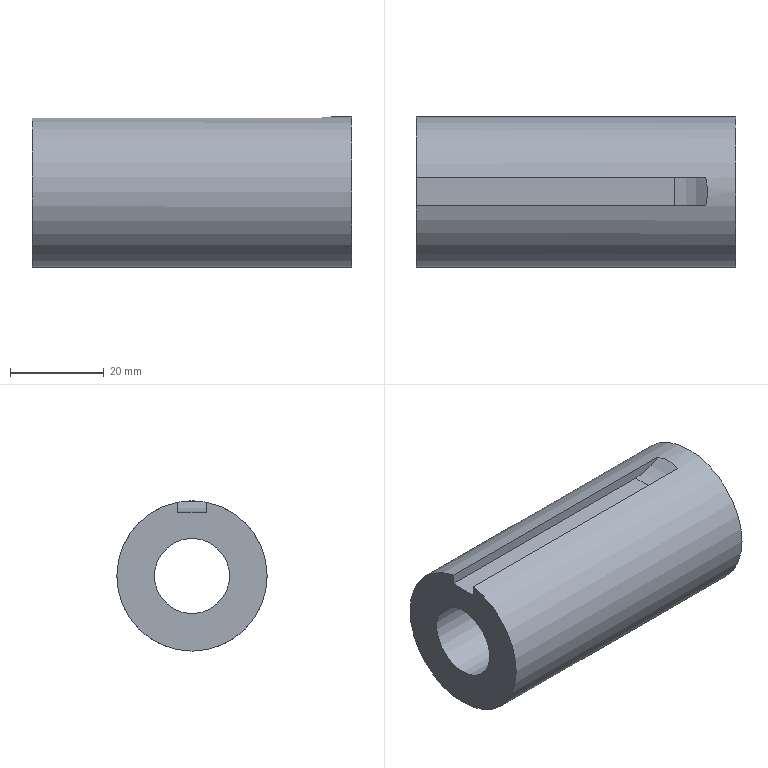Component | NX | SLIDING_SLEEVE | 1 solid | 12 faces | box 68 x 32 x 32 mm | volume 28566 mm3 | plane 7 | cylinder 5 | commonest cylinder face diameters 22 x2 24 x1 32 x1 16 x1
STEP:
#1=CARTESIAN_POINT('',(0.,0.,0.));
#2=DIRECTION('',(0.,0.,1.));
#3=DIRECTION('',(1.,0.,0.));
#4=AXIS2_PLACEMENT_3D('',#1,#2,#3);
#5=CARTESIAN_POINT('',(38.,0.,-8.));
#6=VERTEX_POINT('',#5);
#7=CARTESIAN_POINT('',(38.,0.,0.));
#8=DIRECTION('',(1.,0.,0.));
#9=DIRECTION('',(0.,0.,-1.));
#10=AXIS2_PLACEMENT_3D('',#7,#8,#9);
#11=CIRCLE('',#10,8.);
#12=CARTESIAN_POINT('',(38.,0.,0.));
#13=DIRECTION('',(1.,0.,0.));
#14=DIRECTION('',(0.,0.,-1.));
#15=AXIS2_PLACEMENT_3D('',#12,#13,#14);
#16=PLANE('',#15);
#17=CARTESIAN_POINT('',(0.,0.));
#18=DIRECTION('',(1.,0.));
#19=AXIS2_PLACEMENT_2D('',#17,#18);
#20=CIRCLE('',#19,8.);
#21=(GEOMETRIC_REPRESENTATION_CONTEXT(2)PARAMETRIC_REPRESENTATION_CONTEXT()REPRESENTATION_CONTEXT('',''));
#22=DEFINITIONAL_REPRESENTATION('',(#20),#21);
#23=PCURVE('',#16,#22);
#24=CARTESIAN_POINT('',(38.,0.,0.));
#25=DIRECTION('',(1.,0.,0.));
#26=DIRECTION('',(0.,0.,-1.));
#27=AXIS2_PLACEMENT_3D('',#24,#25,#26);
#28=CYLINDRICAL_SURFACE('',#27,8.);
#29=CARTESIAN_POINT('',(0.,0.));
#30=DIRECTION('',(1.,0.));
#31=VECTOR('',#30,1.);
#32=LINE('',#29,#31);
#33=(GEOMETRIC_REPRESENTATION_CONTEXT(2)PARAMETRIC_REPRESENTATION_CONTEXT()REPRESENTATION_CONTEXT('',''));
#34=DEFINITIONAL_REPRESENTATION('',(#32),#33);
#35=PCURVE('',#28,#34);
#36=SURFACE_CURVE('',#11,(#23,#35),.PCURVE_S1.);
#37=EDGE_CURVE('',#6,#6,#36,.T.);
#38=ORIENTED_EDGE('',*,*,#37,.T.);
#39=EDGE_LOOP('',(#38));
#40=FACE_BOUND('',#39,.T.);
#41=CARTESIAN_POINT('',(38.,3.,15.716));
#42=VERTEX_POINT('',#41);
#43=CARTESIAN_POINT('',(38.,3.,13.5));
#44=VERTEX_POINT('',#43);
#45=CARTESIAN_POINT('',(38.,3.,16.));
#46=DIRECTION('',(0.,0.,-1.));
#47=VECTOR('',#46,1.);
#48=LINE('',#45,#47);
#49=CARTESIAN_POINT('',(-16.,3.));
#50=DIRECTION('',(1.,0.));
#51=VECTOR('',#50,1.);
#52=LINE('',#49,#51);
#53=(GEOMETRIC_REPRESENTATION_CONTEXT(2)PARAMETRIC_REPRESENTATION_CONTEXT()REPRESENTATION_CONTEXT('',''));
#54=DEFINITIONAL_REPRESENTATION('',(#52),#53);
#55=PCURVE('',#16,#54);
#56=CARTESIAN_POINT('',(93.,3.,24.5));
#57=DIRECTION('',(0.,-1.,0.));
#58=DIRECTION('',(0.,0.,-1.));
#59=AXIS2_PLACEMENT_3D('',#56,#57,#58);
#60=PLANE('',#59);
#61=CARTESIAN_POINT('',(8.5,-55.));
#62=DIRECTION('',(1.,0.));
#63=VECTOR('',#62,1.);
#64=LINE('',#61,#63);
#65=(GEOMETRIC_REPRESENTATION_CONTEXT(2)PARAMETRIC_REPRESENTATION_CONTEXT()REPRESENTATION_CONTEXT('',''));
#66=DEFINITIONAL_REPRESENTATION('',(#64),#65);
#67=PCURVE('',#60,#66);
#68=SURFACE_CURVE('',#48,(#55,#67),.PCURVE_S1.);
#69=EDGE_CURVE('',#42,#44,#68,.T.);
#70=ORIENTED_EDGE('',*,*,#69,.F.);
#71=CARTESIAN_POINT('',(38.,-0.,-16.));
#72=VERTEX_POINT('',#71);
#73=CARTESIAN_POINT('',(38.,0.,0.));
#74=DIRECTION('',(1.,0.,0.));
#75=DIRECTION('',(0.,0.,-1.));
#76=AXIS2_PLACEMENT_3D('',#73,#74,#75);
#77=CIRCLE('',#76,16.);
#78=CARTESIAN_POINT('',(0.,0.));
#79=DIRECTION('',(1.,0.));
#80=AXIS2_PLACEMENT_2D('',#78,#79);
#81=CIRCLE('',#80,16.);
#82=(GEOMETRIC_REPRESENTATION_CONTEXT(2)PARAMETRIC_REPRESENTATION_CONTEXT()REPRESENTATION_CONTEXT('',''));
#83=DEFINITIONAL_REPRESENTATION('',(#81),#82);
#84=PCURVE('',#16,#83);
#85=CARTESIAN_POINT('',(38.,0.,0.));
#86=DIRECTION('',(1.,0.,0.));
#87=DIRECTION('',(0.,0.,-1.));
#88=AXIS2_PLACEMENT_3D('',#85,#86,#87);
#89=CYLINDRICAL_SURFACE('',#88,16.);
#90=CARTESIAN_POINT('',(-6.283,0.));
#91=DIRECTION('',(1.,0.));
#92=VECTOR('',#91,1.);
#93=LINE('',#90,#92);
#94=(GEOMETRIC_REPRESENTATION_CONTEXT(2)PARAMETRIC_REPRESENTATION_CONTEXT()REPRESENTATION_CONTEXT('',''));
#95=DEFINITIONAL_REPRESENTATION('',(#93),#94);
#96=PCURVE('',#89,#95);
#97=SURFACE_CURVE('',#77,(#84,#96),.PCURVE_S1.);
#98=EDGE_CURVE('',#72,#42,#97,.T.);
#99=ORIENTED_EDGE('',*,*,#98,.F.);
#100=CARTESIAN_POINT('',(38.,-3.,15.716));
#101=VERTEX_POINT('',#100);
#102=CARTESIAN_POINT('',(38.,0.,0.));
#103=DIRECTION('',(1.,0.,0.));
#104=DIRECTION('',(0.,0.,-1.));
#105=AXIS2_PLACEMENT_3D('',#102,#103,#104);
#106=CIRCLE('',#105,16.);
#107=CARTESIAN_POINT('',(0.,0.));
#108=DIRECTION('',(1.,0.));
#109=AXIS2_PLACEMENT_2D('',#107,#108);
#110=CIRCLE('',#109,16.);
#111=(GEOMETRIC_REPRESENTATION_CONTEXT(2)PARAMETRIC_REPRESENTATION_CONTEXT()REPRESENTATION_CONTEXT('',''));
#112=DEFINITIONAL_REPRESENTATION('',(#110),#111);
#113=PCURVE('',#16,#112);
#114=CARTESIAN_POINT('',(0.,0.));
#115=DIRECTION('',(1.,0.));
#116=VECTOR('',#115,1.);
#117=LINE('',#114,#116);
#118=(GEOMETRIC_REPRESENTATION_CONTEXT(2)PARAMETRIC_REPRESENTATION_CONTEXT()REPRESENTATION_CONTEXT('',''));
#119=DEFINITIONAL_REPRESENTATION('',(#117),#118);
#120=PCURVE('',#89,#119);
#121=SURFACE_CURVE('',#106,(#113,#120),.PCURVE_S1.);
#122=EDGE_CURVE('',#101,#72,#121,.T.);
#123=ORIENTED_EDGE('',*,*,#122,.F.);
#124=CARTESIAN_POINT('',(38.,-3.,13.5));
#125=VERTEX_POINT('',#124);
#126=CARTESIAN_POINT('',(38.,-3.,16.));
#127=DIRECTION('',(0.,0.,-1.));
#128=VECTOR('',#127,1.);
#129=LINE('',#126,#128);
#130=CARTESIAN_POINT('',(-16.,-3.));
#131=DIRECTION('',(1.,0.));
#132=VECTOR('',#131,1.);
#133=LINE('',#130,#132);
#134=(GEOMETRIC_REPRESENTATION_CONTEXT(2)PARAMETRIC_REPRESENTATION_CONTEXT()REPRESENTATION_CONTEXT('',''));
#135=DEFINITIONAL_REPRESENTATION('',(#133),#134);
#136=PCURVE('',#16,#135);
#137=CARTESIAN_POINT('',(93.,-3.,24.5));
#138=DIRECTION('',(0.,-1.,0.));
#139=DIRECTION('',(0.,0.,-1.));
#140=AXIS2_PLACEMENT_3D('',#137,#138,#139);
#141=PLANE('',#140);
#142=CARTESIAN_POINT('',(8.5,-55.));
#143=DIRECTION('',(1.,0.));
#144=VECTOR('',#143,1.);
#145=LINE('',#142,#144);
#146=(GEOMETRIC_REPRESENTATION_CONTEXT(2)PARAMETRIC_REPRESENTATION_CONTEXT()REPRESENTATION_CONTEXT('',''));
#147=DEFINITIONAL_REPRESENTATION('',(#145),#146);
#148=PCURVE('',#141,#147);
#149=SURFACE_CURVE('',#129,(#136,#148),.PCURVE_S1.);
#150=EDGE_CURVE('',#101,#125,#149,.T.);
#151=ORIENTED_EDGE('',*,*,#150,.T.);
#152=CARTESIAN_POINT('',(38.,-3.,13.5));
#153=DIRECTION('',(0.,1.,0.));
#154=VECTOR('',#153,1.);
#155=LINE('',#152,#154);
#156=CARTESIAN_POINT('',(-13.5,-3.));
#157=DIRECTION('',(0.,1.));
#158=VECTOR('',#157,1.);
#159=LINE('',#156,#158);
#160=(GEOMETRIC_REPRESENTATION_CONTEXT(2)PARAMETRIC_REPRESENTATION_CONTEXT()REPRESENTATION_CONTEXT('',''));
#161=DEFINITIONAL_REPRESENTATION('',(#159),#160);
#162=PCURVE('',#16,#161);
#163=CARTESIAN_POINT('',(38.,-3.,13.5));
#164=DIRECTION('',(0.,0.,1.));
#165=DIRECTION('',(1.,0.,0.));
#166=AXIS2_PLACEMENT_3D('',#163,#164,#165);
#167=PLANE('',#166);
#168=CARTESIAN_POINT('',(0.,0.));
#169=DIRECTION('',(0.,1.));
#170=VECTOR('',#169,1.);
#171=LINE('',#168,#170);
#172=(GEOMETRIC_REPRESENTATION_CONTEXT(2)PARAMETRIC_REPRESENTATION_CONTEXT()REPRESENTATION_CONTEXT('',''));
#173=DEFINITIONAL_REPRESENTATION('',(#171),#172);
#174=PCURVE('',#167,#173);
#175=SURFACE_CURVE('',#155,(#162,#174),.PCURVE_S1.);
#176=EDGE_CURVE('',#125,#44,#175,.T.);
#177=ORIENTED_EDGE('',*,*,#176,.T.);
#178=EDGE_LOOP('',(#70,#99,#123,#151,#177));
#179=FACE_BOUND('',#178,.T.);
#180=ADVANCED_FACE('',(#40,#179),#16,.F.);
#181=CARTESIAN_POINT('',(55.,0.,8.));
#182=VERTEX_POINT('',#181);
#183=CARTESIAN_POINT('',(55.,0.,-8.));
#184=VERTEX_POINT('',#183);
#185=CARTESIAN_POINT('',(55.,0.,0.));
#186=DIRECTION('',(-1.,0.,0.));
#187=DIRECTION('',(0.,0.,1.));
#188=AXIS2_PLACEMENT_3D('',#185,#186,#187);
#189=CIRCLE('',#188,8.);
#190=CARTESIAN_POINT('',(55.,12.,0.));
#191=DIRECTION('',(-1.,0.,0.));
#192=DIRECTION('',(0.,0.,1.));
#193=AXIS2_PLACEMENT_3D('',#190,#191,#192);
#194=PLANE('',#193);
#195=CARTESIAN_POINT('',(0.,-12.));
#196=DIRECTION('',(1.,0.));
#197=AXIS2_PLACEMENT_2D('',#195,#196);
#198=CIRCLE('',#197,8.);
#199=(GEOMETRIC_REPRESENTATION_CONTEXT(2)PARAMETRIC_REPRESENTATION_CONTEXT()REPRESENTATION_CONTEXT('',''));
#200=DEFINITIONAL_REPRESENTATION('',(#198),#199);
#201=PCURVE('',#194,#200);
#202=CARTESIAN_POINT('',(3.142,17.));
#203=DIRECTION('',(-1.,0.));
#204=VECTOR('',#203,1.);
#205=LINE('',#202,#204);
#206=(GEOMETRIC_REPRESENTATION_CONTEXT(2)PARAMETRIC_REPRESENTATION_CONTEXT()REPRESENTATION_CONTEXT('',''));
#207=DEFINITIONAL_REPRESENTATION('',(#205),#206);
#208=PCURVE('',#28,#207);
#209=SURFACE_CURVE('',#189,(#201,#208),.PCURVE_S1.);
#210=EDGE_CURVE('',#182,#184,#209,.T.);
#211=ORIENTED_EDGE('',*,*,#210,.T.);
#212=CARTESIAN_POINT('',(55.,0.,0.));
#213=DIRECTION('',(-1.,0.,0.));
#214=DIRECTION('',(0.,0.,1.));
#215=AXIS2_PLACEMENT_3D('',#212,#213,#214);
#216=CIRCLE('',#215,8.);
#217=CARTESIAN_POINT('',(0.,-12.));
#218=DIRECTION('',(1.,0.));
#219=AXIS2_PLACEMENT_2D('',#217,#218);
#220=CIRCLE('',#219,8.);
#221=(GEOMETRIC_REPRESENTATION_CONTEXT(2)PARAMETRIC_REPRESENTATION_CONTEXT()REPRESENTATION_CONTEXT('',''));
#222=DEFINITIONAL_REPRESENTATION('',(#220),#221);
#223=PCURVE('',#194,#222);
#224=CARTESIAN_POINT('',(9.425,17.));
#225=DIRECTION('',(-1.,0.));
#226=VECTOR('',#225,1.);
#227=LINE('',#224,#226);
#228=(GEOMETRIC_REPRESENTATION_CONTEXT(2)PARAMETRIC_REPRESENTATION_CONTEXT()REPRESENTATION_CONTEXT('',''));
#229=DEFINITIONAL_REPRESENTATION('',(#227),#228);
#230=PCURVE('',#28,#229);
#231=SURFACE_CURVE('',#216,(#223,#230),.PCURVE_S1.);
#232=EDGE_CURVE('',#184,#182,#231,.T.);
#233=ORIENTED_EDGE('',*,*,#232,.T.);
#234=EDGE_LOOP('',(#211,#233));
#235=FACE_BOUND('',#234,.T.);
#236=CARTESIAN_POINT('',(55.,0.,-12.));
#237=VERTEX_POINT('',#236);
#238=CARTESIAN_POINT('',(55.,0.,0.));
#239=DIRECTION('',(1.,0.,0.));
#240=DIRECTION('',(0.,0.,-1.));
#241=AXIS2_PLACEMENT_3D('',#238,#239,#240);
#242=CIRCLE('',#241,12.);
#243=CARTESIAN_POINT('',(-12.,-12.));
#244=CARTESIAN_POINT('',(-12.,8.785));
#245=CARTESIAN_POINT('',(6.,-1.608));
#246=CARTESIAN_POINT('',(24.,-12.));
#247=CARTESIAN_POINT('',(6.,-22.392));
#248=CARTESIAN_POINT('',(-12.,-32.785));
#249=CARTESIAN_POINT('',(-12.,-12.));
#250=(BOUNDED_CURVE()B_SPLINE_CURVE(2,(#243,#244,#245,#246,#247,#248,#249),.UNSPECIFIED.,.T.,.F.)B_SPLINE_CURVE_WITH_KNOTS((1,2,2,2,2,1),(-2.094,0.,2.094,4.189,6.283,8.378),.UNSPECIFIED.)CURVE()GEOMETRIC_REPRESENTATION_ITEM()RATIONAL_B_SPLINE_CURVE((1.,0.5,1.,0.5,1.,0.5,1.))REPRESENTATION_ITEM(''));
#251=(GEOMETRIC_REPRESENTATION_CONTEXT(2)PARAMETRIC_REPRESENTATION_CONTEXT()REPRESENTATION_CONTEXT('',''));
#252=DEFINITIONAL_REPRESENTATION('',(#250),#251);
#253=PCURVE('',#194,#252);
#254=CARTESIAN_POINT('',(38.,0.,0.));
#255=DIRECTION('',(1.,0.,0.));
#256=DIRECTION('',(0.,0.,-1.));
#257=AXIS2_PLACEMENT_3D('',#254,#255,#256);
#258=CYLINDRICAL_SURFACE('',#257,12.);
#259=CARTESIAN_POINT('',(0.,17.));
#260=DIRECTION('',(1.,0.));
#261=VECTOR('',#260,1.);
#262=LINE('',#259,#261);
#263=(GEOMETRIC_REPRESENTATION_CONTEXT(2)PARAMETRIC_REPRESENTATION_CONTEXT()REPRESENTATION_CONTEXT('',''));
#264=DEFINITIONAL_REPRESENTATION('',(#262),#263);
#265=PCURVE('',#258,#264);
#266=SURFACE_CURVE('',#242,(#253,#265),.PCURVE_S1.);
#267=EDGE_CURVE('',#237,#237,#266,.T.);
#268=ORIENTED_EDGE('',*,*,#267,.T.);
#269=EDGE_LOOP('',(#268));
#270=FACE_BOUND('',#269,.T.);
#271=ADVANCED_FACE('',(#235,#270),#194,.F.);
#272=ORIENTED_EDGE('',*,*,#267,.T.);
#273=CARTESIAN_POINT('',(89.,0.,-12.));
#274=VERTEX_POINT('',#273);
#275=CARTESIAN_POINT('',(55.,0.,-12.));
#276=CARTESIAN_POINT('',(89.,0.,-12.));
#277=B_SPLINE_CURVE_WITH_KNOTS('',1,(#275,#276),.UNSPECIFIED.,.F.,.F.,(2,2),(17.,51.),.PIECEWISE_BEZIER_KNOTS.);
#278=CARTESIAN_POINT('',(6.283,0.));
#279=DIRECTION('',(0.,1.));
#280=VECTOR('',#279,1.);
#281=LINE('',#278,#280);
#282=(GEOMETRIC_REPRESENTATION_CONTEXT(2)PARAMETRIC_REPRESENTATION_CONTEXT()REPRESENTATION_CONTEXT('',''));
#283=DEFINITIONAL_REPRESENTATION('',(#281),#282);
#284=PCURVE('',#258,#283);
#285=CARTESIAN_POINT('',(0.,0.));
#286=DIRECTION('',(0.,1.));
#287=VECTOR('',#286,1.);
#288=LINE('',#285,#287);
#289=(GEOMETRIC_REPRESENTATION_CONTEXT(2)PARAMETRIC_REPRESENTATION_CONTEXT()REPRESENTATION_CONTEXT('',''));
#290=DEFINITIONAL_REPRESENTATION('',(#288),#289);
#291=PCURVE('',#258,#290);
#292=SEAM_CURVE('',#277,(#284,#291),.PCURVE_S1.);
#293=EDGE_CURVE('',#237,#274,#292,.T.);
#294=ORIENTED_EDGE('',*,*,#293,.T.);
#295=CARTESIAN_POINT('',(89.,0.,0.));
#296=DIRECTION('',(1.,0.,0.));
#297=DIRECTION('',(0.,0.,-1.));
#298=AXIS2_PLACEMENT_3D('',#295,#296,#297);
#299=CIRCLE('',#298,12.);
#300=CARTESIAN_POINT('',(0.,51.));
#301=DIRECTION('',(1.,0.));
#302=VECTOR('',#301,1.);
#303=LINE('',#300,#302);
#304=(GEOMETRIC_REPRESENTATION_CONTEXT(2)PARAMETRIC_REPRESENTATION_CONTEXT()REPRESENTATION_CONTEXT('',''));
#305=DEFINITIONAL_REPRESENTATION('',(#303),#304);
#306=PCURVE('',#258,#305);
#307=CARTESIAN_POINT('',(89.,11.,0.));
#308=DIRECTION('',(1.,0.,0.));
#309=DIRECTION('',(0.,0.,-1.));
#310=AXIS2_PLACEMENT_3D('',#307,#308,#309);
#311=PLANE('',#310);
#312=CARTESIAN_POINT('',(0.,-11.));
#313=DIRECTION('',(1.,0.));
#314=AXIS2_PLACEMENT_2D('',#312,#313);
#315=CIRCLE('',#314,12.);
#316=(GEOMETRIC_REPRESENTATION_CONTEXT(2)PARAMETRIC_REPRESENTATION_CONTEXT()REPRESENTATION_CONTEXT('',''));
#317=DEFINITIONAL_REPRESENTATION('',(#315),#316);
#318=PCURVE('',#311,#317);
#319=SURFACE_CURVE('',#299,(#306,#318),.PCURVE_S1.);
#320=EDGE_CURVE('',#274,#274,#319,.T.);
#321=ORIENTED_EDGE('',*,*,#320,.F.);
#322=ORIENTED_EDGE('',*,*,#293,.F.);
#323=EDGE_LOOP('',(#272,#294,#321,#322));
#324=FACE_BOUND('',#323,.F.);
#325=ADVANCED_FACE('',(#324),#258,.F.);
#326=ORIENTED_EDGE('',*,*,#320,.F.);
#327=EDGE_LOOP('',(#326));
#328=FACE_BOUND('',#327,.T.);
#329=CARTESIAN_POINT('',(89.,0.,-11.));
#330=VERTEX_POINT('',#329);
#331=CARTESIAN_POINT('',(89.,0.,0.));
#332=DIRECTION('',(1.,0.,0.));
#333=DIRECTION('',(0.,0.,-1.));
#334=AXIS2_PLACEMENT_3D('',#331,#332,#333);
#335=CIRCLE('',#334,11.);
#336=CARTESIAN_POINT('',(0.,-11.));
#337=DIRECTION('',(1.,0.));
#338=AXIS2_PLACEMENT_2D('',#336,#337);
#339=CIRCLE('',#338,11.);
#340=(GEOMETRIC_REPRESENTATION_CONTEXT(2)PARAMETRIC_REPRESENTATION_CONTEXT()REPRESENTATION_CONTEXT('',''));
#341=DEFINITIONAL_REPRESENTATION('',(#339),#340);
#342=PCURVE('',#311,#341);
#343=CARTESIAN_POINT('',(38.,0.,0.));
#344=DIRECTION('',(1.,0.,0.));
#345=DIRECTION('',(0.,0.,-1.));
#346=AXIS2_PLACEMENT_3D('',#343,#344,#345);
#347=CYLINDRICAL_SURFACE('',#346,11.);
#348=CARTESIAN_POINT('',(0.,51.));
#349=DIRECTION('',(1.,0.));
#350=VECTOR('',#349,1.);
#351=LINE('',#348,#350);
#352=(GEOMETRIC_REPRESENTATION_CONTEXT(2)PARAMETRIC_REPRESENTATION_CONTEXT()REPRESENTATION_CONTEXT('',''));
#353=DEFINITIONAL_REPRESENTATION('',(#351),#352);
#354=PCURVE('',#347,#353);
#355=SURFACE_CURVE('',#335,(#342,#354),.PCURVE_S1.);
#356=EDGE_CURVE('',#330,#330,#355,.T.);
#357=ORIENTED_EDGE('',*,*,#356,.T.);
#358=EDGE_LOOP('',(#357));
#359=FACE_BOUND('',#358,.T.);
#360=ADVANCED_FACE('',(#328,#359),#311,.F.);
#361=ORIENTED_EDGE('',*,*,#356,.T.);
#362=CARTESIAN_POINT('',(106.,0.,-11.));
#363=VERTEX_POINT('',#362);
#364=CARTESIAN_POINT('',(89.,0.,-11.));
#365=CARTESIAN_POINT('',(106.,0.,-11.));
#366=B_SPLINE_CURVE_WITH_KNOTS('',1,(#364,#365),.UNSPECIFIED.,.F.,.F.,(2,2),(51.,68.),.PIECEWISE_BEZIER_KNOTS.);
#367=CARTESIAN_POINT('',(6.283,0.));
#368=DIRECTION('',(0.,1.));
#369=VECTOR('',#368,1.);
#370=LINE('',#367,#369);
#371=(GEOMETRIC_REPRESENTATION_CONTEXT(2)PARAMETRIC_REPRESENTATION_CONTEXT()REPRESENTATION_CONTEXT('',''));
#372=DEFINITIONAL_REPRESENTATION('',(#370),#371);
#373=PCURVE('',#347,#372);
#374=CARTESIAN_POINT('',(0.,0.));
#375=DIRECTION('',(0.,1.));
#376=VECTOR('',#375,1.);
#377=LINE('',#374,#376);
#378=(GEOMETRIC_REPRESENTATION_CONTEXT(2)PARAMETRIC_REPRESENTATION_CONTEXT()REPRESENTATION_CONTEXT('',''));
#379=DEFINITIONAL_REPRESENTATION('',(#377),#378);
#380=PCURVE('',#347,#379);
#381=SEAM_CURVE('',#366,(#373,#380),.PCURVE_S1.);
#382=EDGE_CURVE('',#330,#363,#381,.T.);
#383=ORIENTED_EDGE('',*,*,#382,.T.);
#384=CARTESIAN_POINT('',(106.,0.,0.));
#385=DIRECTION('',(1.,0.,0.));
#386=DIRECTION('',(0.,0.,-1.));
#387=AXIS2_PLACEMENT_3D('',#384,#385,#386);
#388=CIRCLE('',#387,11.);
#389=CARTESIAN_POINT('',(0.,68.));
#390=DIRECTION('',(1.,0.));
#391=VECTOR('',#390,1.);
#392=LINE('',#389,#391);
#393=(GEOMETRIC_REPRESENTATION_CONTEXT(2)PARAMETRIC_REPRESENTATION_CONTEXT()REPRESENTATION_CONTEXT('',''));
#394=DEFINITIONAL_REPRESENTATION('',(#392),#393);
#395=PCURVE('',#347,#394);
#396=CARTESIAN_POINT('',(106.,16.,0.));
#397=DIRECTION('',(-1.,0.,0.));
#398=DIRECTION('',(0.,0.,1.));
#399=AXIS2_PLACEMENT_3D('',#396,#397,#398);
#400=PLANE('',#399);
#401=CARTESIAN_POINT('',(-11.,-16.));
#402=CARTESIAN_POINT('',(-11.,3.053));
#403=CARTESIAN_POINT('',(5.5,-6.474));
#404=CARTESIAN_POINT('',(22.,-16.));
#405=CARTESIAN_POINT('',(5.5,-25.526));
#406=CARTESIAN_POINT('',(-11.,-35.053));
#407=CARTESIAN_POINT('',(-11.,-16.));
#408=(BOUNDED_CURVE()B_SPLINE_CURVE(2,(#401,#402,#403,#404,#405,#406,#407),.UNSPECIFIED.,.T.,.F.)B_SPLINE_CURVE_WITH_KNOTS((1,2,2,2,2,1),(-2.094,0.,2.094,4.189,6.283,8.378),.UNSPECIFIED.)CURVE()GEOMETRIC_REPRESENTATION_ITEM()RATIONAL_B_SPLINE_CURVE((1.,0.5,1.,0.5,1.,0.5,1.))REPRESENTATION_ITEM(''));
#409=(GEOMETRIC_REPRESENTATION_CONTEXT(2)PARAMETRIC_REPRESENTATION_CONTEXT()REPRESENTATION_CONTEXT('',''));
#410=DEFINITIONAL_REPRESENTATION('',(#408),#409);
#411=PCURVE('',#400,#410);
#412=SURFACE_CURVE('',#388,(#395,#411),.PCURVE_S1.);
#413=EDGE_CURVE('',#363,#363,#412,.T.);
#414=ORIENTED_EDGE('',*,*,#413,.F.);
#415=ORIENTED_EDGE('',*,*,#382,.F.);
#416=EDGE_LOOP('',(#361,#383,#414,#415));
#417=FACE_BOUND('',#416,.F.);
#418=ADVANCED_FACE('',(#417),#347,.F.);
#419=ORIENTED_EDGE('',*,*,#413,.F.);
#420=EDGE_LOOP('',(#419));
#421=FACE_BOUND('',#420,.T.);
#422=CARTESIAN_POINT('',(106.,0.,-16.));
#423=VERTEX_POINT('',#422);
#424=CARTESIAN_POINT('',(106.,0.,0.));
#425=DIRECTION('',(1.,0.,0.));
#426=DIRECTION('',(0.,0.,-1.));
#427=AXIS2_PLACEMENT_3D('',#424,#425,#426);
#428=CIRCLE('',#427,16.);
#429=CARTESIAN_POINT('',(-16.,-16.));
#430=CARTESIAN_POINT('',(-16.,11.713));
#431=CARTESIAN_POINT('',(8.,-2.144));
#432=CARTESIAN_POINT('',(32.,-16.));
#433=CARTESIAN_POINT('',(8.,-29.856));
#434=CARTESIAN_POINT('',(-16.,-43.713));
#435=CARTESIAN_POINT('',(-16.,-16.));
#436=(BOUNDED_CURVE()B_SPLINE_CURVE(2,(#429,#430,#431,#432,#433,#434,#435),.UNSPECIFIED.,.T.,.F.)B_SPLINE_CURVE_WITH_KNOTS((1,2,2,2,2,1),(-2.094,0.,2.094,4.189,6.283,8.378),.UNSPECIFIED.)CURVE()GEOMETRIC_REPRESENTATION_ITEM()RATIONAL_B_SPLINE_CURVE((1.,0.5,1.,0.5,1.,0.5,1.))REPRESENTATION_ITEM(''));
#437=(GEOMETRIC_REPRESENTATION_CONTEXT(2)PARAMETRIC_REPRESENTATION_CONTEXT()REPRESENTATION_CONTEXT('',''));
#438=DEFINITIONAL_REPRESENTATION('',(#436),#437);
#439=PCURVE('',#400,#438);
#440=CARTESIAN_POINT('',(0.,68.));
#441=DIRECTION('',(1.,0.));
#442=VECTOR('',#441,1.);
#443=LINE('',#440,#442);
#444=(GEOMETRIC_REPRESENTATION_CONTEXT(2)PARAMETRIC_REPRESENTATION_CONTEXT()REPRESENTATION_CONTEXT('',''));
#445=DEFINITIONAL_REPRESENTATION('',(#443),#444);
#446=PCURVE('',#89,#445);
#447=SURFACE_CURVE('',#428,(#439,#446),.PCURVE_S1.);
#448=EDGE_CURVE('',#423,#423,#447,.T.);
#449=ORIENTED_EDGE('',*,*,#448,.T.);
#450=EDGE_LOOP('',(#449));
#451=FACE_BOUND('',#450,.T.);
#452=ADVANCED_FACE('',(#421,#451),#400,.F.);
#453=ORIENTED_EDGE('',*,*,#448,.F.);
#454=CARTESIAN_POINT('',(38.,-0.,-16.));
#455=CARTESIAN_POINT('',(106.,-0.,-16.));
#456=B_SPLINE_CURVE_WITH_KNOTS('',1,(#454,#455),.UNSPECIFIED.,.F.,.F.,(2,2),(0.,68.),.PIECEWISE_BEZIER_KNOTS.);
#457=CARTESIAN_POINT('',(0.,0.));
#458=DIRECTION('',(0.,1.));
#459=VECTOR('',#458,1.);
#460=LINE('',#457,#459);
#461=(GEOMETRIC_REPRESENTATION_CONTEXT(2)PARAMETRIC_REPRESENTATION_CONTEXT()REPRESENTATION_CONTEXT('',''));
#462=DEFINITIONAL_REPRESENTATION('',(#460),#461);
#463=PCURVE('',#89,#462);
#464=CARTESIAN_POINT('',(6.283,0.));
#465=DIRECTION('',(0.,1.));
#466=VECTOR('',#465,1.);
#467=LINE('',#464,#466);
#468=(GEOMETRIC_REPRESENTATION_CONTEXT(2)PARAMETRIC_REPRESENTATION_CONTEXT()REPRESENTATION_CONTEXT('',''));
#469=DEFINITIONAL_REPRESENTATION('',(#467),#468);
#470=PCURVE('',#89,#469);
#471=SEAM_CURVE('',#456,(#463,#470),.PCURVE_S1.);
#472=EDGE_CURVE('',#72,#423,#471,.T.);
#473=ORIENTED_EDGE('',*,*,#472,.F.);
#474=ORIENTED_EDGE('',*,*,#98,.T.);
#475=CARTESIAN_POINT('',(99.622,3.,15.716));
#476=VERTEX_POINT('',#475);
#477=CARTESIAN_POINT('',(38.,3.,15.716));
#478=DIRECTION('',(-1.,0.,0.));
#479=VECTOR('',#478,1.);
#480=LINE('',#477,#479);
#481=CARTESIAN_POINT('',(2.953,0.));
#482=DIRECTION('',(0.,-1.));
#483=VECTOR('',#482,1.);
#484=LINE('',#481,#483);
#485=(GEOMETRIC_REPRESENTATION_CONTEXT(2)PARAMETRIC_REPRESENTATION_CONTEXT()REPRESENTATION_CONTEXT('',''));
#486=DEFINITIONAL_REPRESENTATION('',(#484),#485);
#487=PCURVE('',#89,#486);
#488=CARTESIAN_POINT('',(8.784,-55.));
#489=DIRECTION('',(0.,-1.));
#490=VECTOR('',#489,1.);
#491=LINE('',#488,#490);
#492=(GEOMETRIC_REPRESENTATION_CONTEXT(2)PARAMETRIC_REPRESENTATION_CONTEXT()REPRESENTATION_CONTEXT('',''));
#493=DEFINITIONAL_REPRESENTATION('',(#491),#492);
#494=PCURVE('',#60,#493);
#495=SURFACE_CURVE('',#480,(#487,#494),.PCURVE_S1.);
#496=EDGE_CURVE('',#476,#42,#495,.T.);
#497=ORIENTED_EDGE('',*,*,#496,.F.);
#498=CARTESIAN_POINT('',(99.622,-3.,15.716));
#499=VERTEX_POINT('',#498);
#500=CARTESIAN_POINT('',(99.622,-3.,15.716));
#501=CARTESIAN_POINT('',(100.116,-1.047,16.089));
#502=CARTESIAN_POINT('',(100.116,1.048,16.089));
#503=CARTESIAN_POINT('',(99.622,3.,15.716));
#504=B_SPLINE_CURVE_WITH_KNOTS('',3,(#500,#501,#502,#503),.UNSPECIFIED.,.F.,.F.,(4,4),(0.,1.),.PIECEWISE_BEZIER_KNOTS.);
#505=CARTESIAN_POINT('',(3.33,61.622));
#506=CARTESIAN_POINT('',(3.325,61.644));
#507=CARTESIAN_POINT('',(3.313,61.687));
#508=CARTESIAN_POINT('',(3.296,61.745));
#509=CARTESIAN_POINT('',(3.279,61.797));
#510=CARTESIAN_POINT('',(3.262,61.843));
#511=CARTESIAN_POINT('',(3.245,61.883));
#512=CARTESIAN_POINT('',(3.228,61.917));
#513=CARTESIAN_POINT('',(3.211,61.944));
#514=CARTESIAN_POINT('',(3.193,61.966));
#515=CARTESIAN_POINT('',(3.176,61.981));
#516=CARTESIAN_POINT('',(3.159,61.99));
#517=CARTESIAN_POINT('',(3.142,61.993));
#518=CARTESIAN_POINT('',(3.124,61.99));
#519=CARTESIAN_POINT('',(3.107,61.981));
#520=CARTESIAN_POINT('',(3.09,61.966));
#521=CARTESIAN_POINT('',(3.073,61.944));
#522=CARTESIAN_POINT('',(3.055,61.917));
#523=CARTESIAN_POINT('',(3.038,61.883));
#524=CARTESIAN_POINT('',(3.021,61.843));
#525=CARTESIAN_POINT('',(3.004,61.797));
#526=CARTESIAN_POINT('',(2.987,61.745));
#527=CARTESIAN_POINT('',(2.97,61.687));
#528=CARTESIAN_POINT('',(2.959,61.644));
#529=CARTESIAN_POINT('',(2.953,61.622));
#530=B_SPLINE_CURVE_WITH_KNOTS('',3,(#505,#506,#507,#508,#509,#510,#511,#512,#513,#514,#515,#516,#517,#518,#519,#520,#521,#522,#523,#524,#525,#526,#527,#528,#529),.UNSPECIFIED.,.F.,.F.,(4,1,1,1,1,1,1,1,1,1,1,1,1,1,1,1,1,1,1,1,1,1,4),(0.,0.04545,0.09091,0.1364,0.1818,0.2273,0.2727,0.3182,0.3636,0.4091,0.4545,0.5,0.5455,0.5909,0.6364,0.6818,0.7273,0.7727,0.8182,0.8636,0.9091,0.9545,1.),.QUASI_UNIFORM_KNOTS.);
#531=(GEOMETRIC_REPRESENTATION_CONTEXT(2)PARAMETRIC_REPRESENTATION_CONTEXT()REPRESENTATION_CONTEXT('',''));
#532=DEFINITIONAL_REPRESENTATION('',(#530),#531);
#533=PCURVE('',#89,#532);
#534=CARTESIAN_POINT('',(93.,-3.,24.5));
#535=DIRECTION('',(0.,1.,0.));
#536=DIRECTION('',(0.,0.,1.));
#537=AXIS2_PLACEMENT_3D('',#534,#535,#536);
#538=CYLINDRICAL_SURFACE('',#537,11.);
#539=CARTESIAN_POINT('',(2.496,0.));
#540=CARTESIAN_POINT('',(2.493,0.08876));
#541=CARTESIAN_POINT('',(2.488,0.2669));
#542=CARTESIAN_POINT('',(2.482,0.5356));
#543=CARTESIAN_POINT('',(2.476,0.8059));
#544=CARTESIAN_POINT('',(2.47,1.077));
#545=CARTESIAN_POINT('',(2.466,1.35));
#546=CARTESIAN_POINT('',(2.462,1.624));
#547=CARTESIAN_POINT('',(2.459,1.898));
#548=CARTESIAN_POINT('',(2.456,2.173));
#549=CARTESIAN_POINT('',(2.455,2.448));
#550=CARTESIAN_POINT('',(2.454,2.724));
#551=CARTESIAN_POINT('',(2.453,3.));
#552=CARTESIAN_POINT('',(2.454,3.276));
#553=CARTESIAN_POINT('',(2.455,3.552));
#554=CARTESIAN_POINT('',(2.456,3.827));
#555=CARTESIAN_POINT('',(2.459,4.102));
#556=CARTESIAN_POINT('',(2.462,4.377));
#557=CARTESIAN_POINT('',(2.466,4.65));
#558=CARTESIAN_POINT('',(2.47,4.923));
#559=CARTESIAN_POINT('',(2.476,5.194));
#560=CARTESIAN_POINT('',(2.482,5.464));
#561=CARTESIAN_POINT('',(2.488,5.733));
#562=CARTESIAN_POINT('',(2.493,5.911));
#563=CARTESIAN_POINT('',(2.496,6.));
#564=B_SPLINE_CURVE_WITH_KNOTS('',3,(#539,#540,#541,#542,#543,#544,#545,#546,#547,#548,#549,#550,#551,#552,#553,#554,#555,#556,#557,#558,#559,#560,#561,#562,#563),.UNSPECIFIED.,.F.,.F.,(4,1,1,1,1,1,1,1,1,1,1,1,1,1,1,1,1,1,1,1,1,1,4),(0.,0.04545,0.09091,0.1364,0.1818,0.2273,0.2727,0.3182,0.3636,0.4091,0.4545,0.5,0.5455,0.5909,0.6364,0.6818,0.7273,0.7727,0.8182,0.8636,0.9091,0.9545,1.),.QUASI_UNIFORM_KNOTS.);
#565=(GEOMETRIC_REPRESENTATION_CONTEXT(2)PARAMETRIC_REPRESENTATION_CONTEXT()REPRESENTATION_CONTEXT('',''));
#566=DEFINITIONAL_REPRESENTATION('',(#564),#565);
#567=PCURVE('',#538,#566);
#568=SURFACE_CURVE('',#504,(#533,#567),.PCURVE_S1.);
#569=EDGE_CURVE('',#499,#476,#568,.T.);
#570=ORIENTED_EDGE('',*,*,#569,.F.);
#571=CARTESIAN_POINT('',(38.,-3.,15.716));
#572=DIRECTION('',(-1.,0.,0.));
#573=VECTOR('',#572,1.);
#574=LINE('',#571,#573);
#575=CARTESIAN_POINT('',(3.33,0.));
#576=DIRECTION('',(0.,-1.));
#577=VECTOR('',#576,1.);
#578=LINE('',#575,#577);
#579=(GEOMETRIC_REPRESENTATION_CONTEXT(2)PARAMETRIC_REPRESENTATION_CONTEXT()REPRESENTATION_CONTEXT('',''));
#580=DEFINITIONAL_REPRESENTATION('',(#578),#579);
#581=PCURVE('',#89,#580);
#582=CARTESIAN_POINT('',(8.784,-55.));
#583=DIRECTION('',(0.,-1.));
#584=VECTOR('',#583,1.);
#585=LINE('',#582,#584);
#586=(GEOMETRIC_REPRESENTATION_CONTEXT(2)PARAMETRIC_REPRESENTATION_CONTEXT()REPRESENTATION_CONTEXT('',''));
#587=DEFINITIONAL_REPRESENTATION('',(#585),#586);
#588=PCURVE('',#141,#587);
#589=SURFACE_CURVE('',#574,(#581,#588),.PCURVE_S1.);
#590=EDGE_CURVE('',#499,#101,#589,.T.);
#591=ORIENTED_EDGE('',*,*,#590,.T.);
#592=ORIENTED_EDGE('',*,*,#122,.T.);
#593=ORIENTED_EDGE('',*,*,#472,.T.);
#594=EDGE_LOOP('',(#453,#473,#474,#497,#570,#591,#592,#593));
#595=FACE_BOUND('',#594,.T.);
#596=ADVANCED_FACE('',(#595),#89,.T.);
#597=ORIENTED_EDGE('',*,*,#37,.T.);
#598=CARTESIAN_POINT('',(38.,0.,-8.));
#599=CARTESIAN_POINT('',(55.,0.,-8.));
#600=B_SPLINE_CURVE_WITH_KNOTS('',1,(#598,#599),.UNSPECIFIED.,.F.,.F.,(2,2),(0.,17.),.PIECEWISE_BEZIER_KNOTS.);
#601=CARTESIAN_POINT('',(6.283,0.));
#602=DIRECTION('',(0.,1.));
#603=VECTOR('',#602,1.);
#604=LINE('',#601,#603);
#605=(GEOMETRIC_REPRESENTATION_CONTEXT(2)PARAMETRIC_REPRESENTATION_CONTEXT()REPRESENTATION_CONTEXT('',''));
#606=DEFINITIONAL_REPRESENTATION('',(#604),#605);
#607=PCURVE('',#28,#606);
#608=CARTESIAN_POINT('',(0.,0.));
#609=DIRECTION('',(0.,1.));
#610=VECTOR('',#609,1.);
#611=LINE('',#608,#610);
#612=(GEOMETRIC_REPRESENTATION_CONTEXT(2)PARAMETRIC_REPRESENTATION_CONTEXT()REPRESENTATION_CONTEXT('',''));
#613=DEFINITIONAL_REPRESENTATION('',(#611),#612);
#614=PCURVE('',#28,#613);
#615=SEAM_CURVE('',#600,(#607,#614),.PCURVE_S1.);
#616=EDGE_CURVE('',#6,#184,#615,.T.);
#617=ORIENTED_EDGE('',*,*,#616,.T.);
#618=ORIENTED_EDGE('',*,*,#232,.T.);
#619=ORIENTED_EDGE('',*,*,#210,.T.);
#620=ORIENTED_EDGE('',*,*,#616,.F.);
#621=EDGE_LOOP('',(#597,#617,#618,#619,#620));
#622=FACE_BOUND('',#621,.F.);
#623=ADVANCED_FACE('',(#622),#28,.F.);
#624=CARTESIAN_POINT('',(93.,3.,13.5));
#625=VERTEX_POINT('',#624);
#626=CARTESIAN_POINT('',(93.,-3.,13.5));
#627=VERTEX_POINT('',#626);
#628=CARTESIAN_POINT('',(93.,-3.,13.5));
#629=DIRECTION('',(0.,-1.,0.));
#630=VECTOR('',#629,1.);
#631=LINE('',#628,#630);
#632=CARTESIAN_POINT('',(3.142,0.));
#633=DIRECTION('',(0.,-1.));
#634=VECTOR('',#633,1.);
#635=LINE('',#632,#634);
#636=(GEOMETRIC_REPRESENTATION_CONTEXT(2)PARAMETRIC_REPRESENTATION_CONTEXT()REPRESENTATION_CONTEXT('',''));
#637=DEFINITIONAL_REPRESENTATION('',(#635),#636);
#638=PCURVE('',#538,#637);
#639=CARTESIAN_POINT('',(55.,0.));
#640=DIRECTION('',(0.,-1.));
#641=VECTOR('',#640,1.);
#642=LINE('',#639,#641);
#643=(GEOMETRIC_REPRESENTATION_CONTEXT(2)PARAMETRIC_REPRESENTATION_CONTEXT()REPRESENTATION_CONTEXT('',''));
#644=DEFINITIONAL_REPRESENTATION('',(#642),#643);
#645=PCURVE('',#167,#644);
#646=SURFACE_CURVE('',#631,(#638,#645),.PCURVE_S1.);
#647=EDGE_CURVE('',#625,#627,#646,.T.);
#648=ORIENTED_EDGE('',*,*,#647,.F.);
#649=CARTESIAN_POINT('',(93.,3.,24.5));
#650=DIRECTION('',(0.,1.,0.));
#651=DIRECTION('',(0.,0.,1.));
#652=AXIS2_PLACEMENT_3D('',#649,#650,#651);
#653=CIRCLE('',#652,11.);
#654=CARTESIAN_POINT('',(0.,6.));
#655=DIRECTION('',(1.,0.));
#656=VECTOR('',#655,1.);
#657=LINE('',#654,#656);
#658=(GEOMETRIC_REPRESENTATION_CONTEXT(2)PARAMETRIC_REPRESENTATION_CONTEXT()REPRESENTATION_CONTEXT('',''));
#659=DEFINITIONAL_REPRESENTATION('',(#657),#658);
#660=PCURVE('',#538,#659);
#661=CARTESIAN_POINT('',(-11.,0.));
#662=CARTESIAN_POINT('',(-11.,19.053));
#663=CARTESIAN_POINT('',(5.5,9.526));
#664=CARTESIAN_POINT('',(22.,0.));
#665=CARTESIAN_POINT('',(5.5,-9.526));
#666=CARTESIAN_POINT('',(-11.,-19.053));
#667=CARTESIAN_POINT('',(-11.,0.));
#668=(BOUNDED_CURVE()B_SPLINE_CURVE(2,(#661,#662,#663,#664,#665,#666,#667),.UNSPECIFIED.,.T.,.F.)B_SPLINE_CURVE_WITH_KNOTS((1,2,2,2,2,1),(-2.094,0.,2.094,4.189,6.283,8.378),.UNSPECIFIED.)CURVE()GEOMETRIC_REPRESENTATION_ITEM()RATIONAL_B_SPLINE_CURVE((1.,0.5,1.,0.5,1.,0.5,1.))REPRESENTATION_ITEM(''));
#669=(GEOMETRIC_REPRESENTATION_CONTEXT(2)PARAMETRIC_REPRESENTATION_CONTEXT()REPRESENTATION_CONTEXT('',''));
#670=DEFINITIONAL_REPRESENTATION('',(#668),#669);
#671=PCURVE('',#60,#670);
#672=SURFACE_CURVE('',#653,(#660,#671),.PCURVE_S1.);
#673=EDGE_CURVE('',#476,#625,#672,.T.);
#674=ORIENTED_EDGE('',*,*,#673,.F.);
#675=ORIENTED_EDGE('',*,*,#569,.F.);
#676=CARTESIAN_POINT('',(93.,-3.,24.5));
#677=DIRECTION('',(0.,1.,0.));
#678=DIRECTION('',(0.,0.,1.));
#679=AXIS2_PLACEMENT_3D('',#676,#677,#678);
#680=CIRCLE('',#679,11.);
#681=CARTESIAN_POINT('',(0.,0.));
#682=DIRECTION('',(1.,0.));
#683=VECTOR('',#682,1.);
#684=LINE('',#681,#683);
#685=(GEOMETRIC_REPRESENTATION_CONTEXT(2)PARAMETRIC_REPRESENTATION_CONTEXT()REPRESENTATION_CONTEXT('',''));
#686=DEFINITIONAL_REPRESENTATION('',(#684),#685);
#687=PCURVE('',#538,#686);
#688=CARTESIAN_POINT('',(-11.,0.));
#689=CARTESIAN_POINT('',(-11.,19.053));
#690=CARTESIAN_POINT('',(5.5,9.526));
#691=CARTESIAN_POINT('',(22.,0.));
#692=CARTESIAN_POINT('',(5.5,-9.526));
#693=CARTESIAN_POINT('',(-11.,-19.053));
#694=CARTESIAN_POINT('',(-11.,0.));
#695=(BOUNDED_CURVE()B_SPLINE_CURVE(2,(#688,#689,#690,#691,#692,#693,#694),.UNSPECIFIED.,.T.,.F.)B_SPLINE_CURVE_WITH_KNOTS((1,2,2,2,2,1),(-2.094,0.,2.094,4.189,6.283,8.378),.UNSPECIFIED.)CURVE()GEOMETRIC_REPRESENTATION_ITEM()RATIONAL_B_SPLINE_CURVE((1.,0.5,1.,0.5,1.,0.5,1.))REPRESENTATION_ITEM(''));
#696=(GEOMETRIC_REPRESENTATION_CONTEXT(2)PARAMETRIC_REPRESENTATION_CONTEXT()REPRESENTATION_CONTEXT('',''));
#697=DEFINITIONAL_REPRESENTATION('',(#695),#696);
#698=PCURVE('',#141,#697);
#699=SURFACE_CURVE('',#680,(#687,#698),.PCURVE_S1.);
#700=EDGE_CURVE('',#499,#627,#699,.T.);
#701=ORIENTED_EDGE('',*,*,#700,.T.);
#702=EDGE_LOOP('',(#648,#674,#675,#701));
#703=FACE_BOUND('',#702,.F.);
#704=ADVANCED_FACE('',(#703),#538,.F.);
#705=ORIENTED_EDGE('',*,*,#700,.T.);
#706=CARTESIAN_POINT('',(38.,-3.,13.5));
#707=DIRECTION('',(-1.,0.,0.));
#708=VECTOR('',#707,1.);
#709=LINE('',#706,#708);
#710=CARTESIAN_POINT('',(11.,-55.));
#711=DIRECTION('',(0.,-1.));
#712=VECTOR('',#711,1.);
#713=LINE('',#710,#712);
#714=(GEOMETRIC_REPRESENTATION_CONTEXT(2)PARAMETRIC_REPRESENTATION_CONTEXT()REPRESENTATION_CONTEXT('',''));
#715=DEFINITIONAL_REPRESENTATION('',(#713),#714);
#716=PCURVE('',#141,#715);
#717=CARTESIAN_POINT('',(0.,0.));
#718=DIRECTION('',(-1.,0.));
#719=VECTOR('',#718,1.);
#720=LINE('',#717,#719);
#721=(GEOMETRIC_REPRESENTATION_CONTEXT(2)PARAMETRIC_REPRESENTATION_CONTEXT()REPRESENTATION_CONTEXT('',''));
#722=DEFINITIONAL_REPRESENTATION('',(#720),#721);
#723=PCURVE('',#167,#722);
#724=SURFACE_CURVE('',#709,(#716,#723),.PCURVE_S1.);
#725=EDGE_CURVE('',#627,#125,#724,.T.);
#726=ORIENTED_EDGE('',*,*,#725,.T.);
#727=ORIENTED_EDGE('',*,*,#150,.F.);
#728=ORIENTED_EDGE('',*,*,#590,.F.);
#729=EDGE_LOOP('',(#705,#726,#727,#728));
#730=FACE_BOUND('',#729,.T.);
#731=ADVANCED_FACE('',(#730),#141,.F.);
#732=ORIENTED_EDGE('',*,*,#496,.T.);
#733=ORIENTED_EDGE('',*,*,#69,.T.);
#734=CARTESIAN_POINT('',(38.,3.,13.5));
#735=DIRECTION('',(-1.,0.,0.));
#736=VECTOR('',#735,1.);
#737=LINE('',#734,#736);
#738=CARTESIAN_POINT('',(11.,-55.));
#739=DIRECTION('',(0.,-1.));
#740=VECTOR('',#739,1.);
#741=LINE('',#738,#740);
#742=(GEOMETRIC_REPRESENTATION_CONTEXT(2)PARAMETRIC_REPRESENTATION_CONTEXT()REPRESENTATION_CONTEXT('',''));
#743=DEFINITIONAL_REPRESENTATION('',(#741),#742);
#744=PCURVE('',#60,#743);
#745=CARTESIAN_POINT('',(0.,6.));
#746=DIRECTION('',(-1.,0.));
#747=VECTOR('',#746,1.);
#748=LINE('',#745,#747);
#749=(GEOMETRIC_REPRESENTATION_CONTEXT(2)PARAMETRIC_REPRESENTATION_CONTEXT()REPRESENTATION_CONTEXT('',''));
#750=DEFINITIONAL_REPRESENTATION('',(#748),#749);
#751=PCURVE('',#167,#750);
#752=SURFACE_CURVE('',#737,(#744,#751),.PCURVE_S1.);
#753=EDGE_CURVE('',#625,#44,#752,.T.);
#754=ORIENTED_EDGE('',*,*,#753,.F.);
#755=ORIENTED_EDGE('',*,*,#673,.F.);
#756=EDGE_LOOP('',(#732,#733,#754,#755));
#757=FACE_BOUND('',#756,.T.);
#758=ADVANCED_FACE('',(#757),#60,.T.);
#759=ORIENTED_EDGE('',*,*,#753,.T.);
#760=ORIENTED_EDGE('',*,*,#176,.F.);
#761=ORIENTED_EDGE('',*,*,#725,.F.);
#762=ORIENTED_EDGE('',*,*,#647,.F.);
#763=EDGE_LOOP('',(#759,#760,#761,#762));
#764=FACE_BOUND('',#763,.T.);
#765=ADVANCED_FACE('',(#764),#167,.T.);
#766=CLOSED_SHELL('',(#180,#271,#325,#360,#418,#452,#596,#623,#704,#731,#758,#765));
#767=MANIFOLD_SOLID_BREP('',#766);
#768=(LENGTH_UNIT()NAMED_UNIT(*)SI_UNIT(.MILLI.,.METRE.));
#769=UNCERTAINTY_MEASURE_WITH_UNIT(LENGTH_MEASURE(0.001),#768,'','');
#770=(NAMED_UNIT(*)PLANE_ANGLE_UNIT()SI_UNIT($,.RADIAN.));
#771=(NAMED_UNIT(*)SI_UNIT($,.STERADIAN.)SOLID_ANGLE_UNIT());
#772=(GEOMETRIC_REPRESENTATION_CONTEXT(3)GLOBAL_UNCERTAINTY_ASSIGNED_CONTEXT((#769))GLOBAL_UNIT_ASSIGNED_CONTEXT((#768,#770,#771))REPRESENTATION_CONTEXT('',''));
#773=ADVANCED_BREP_SHAPE_REPRESENTATION('',(#4,#767),#772);